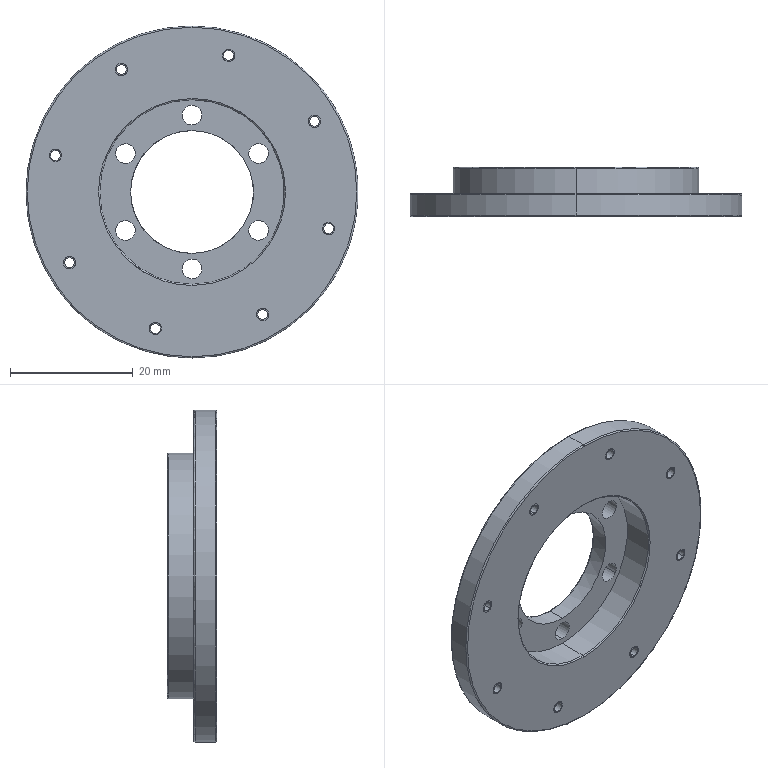CAM job | Mastercam | mm | 1 operations | part box 54 x 8 x 54
1. Drill/Counterbore | 7 - 4 倒角刀